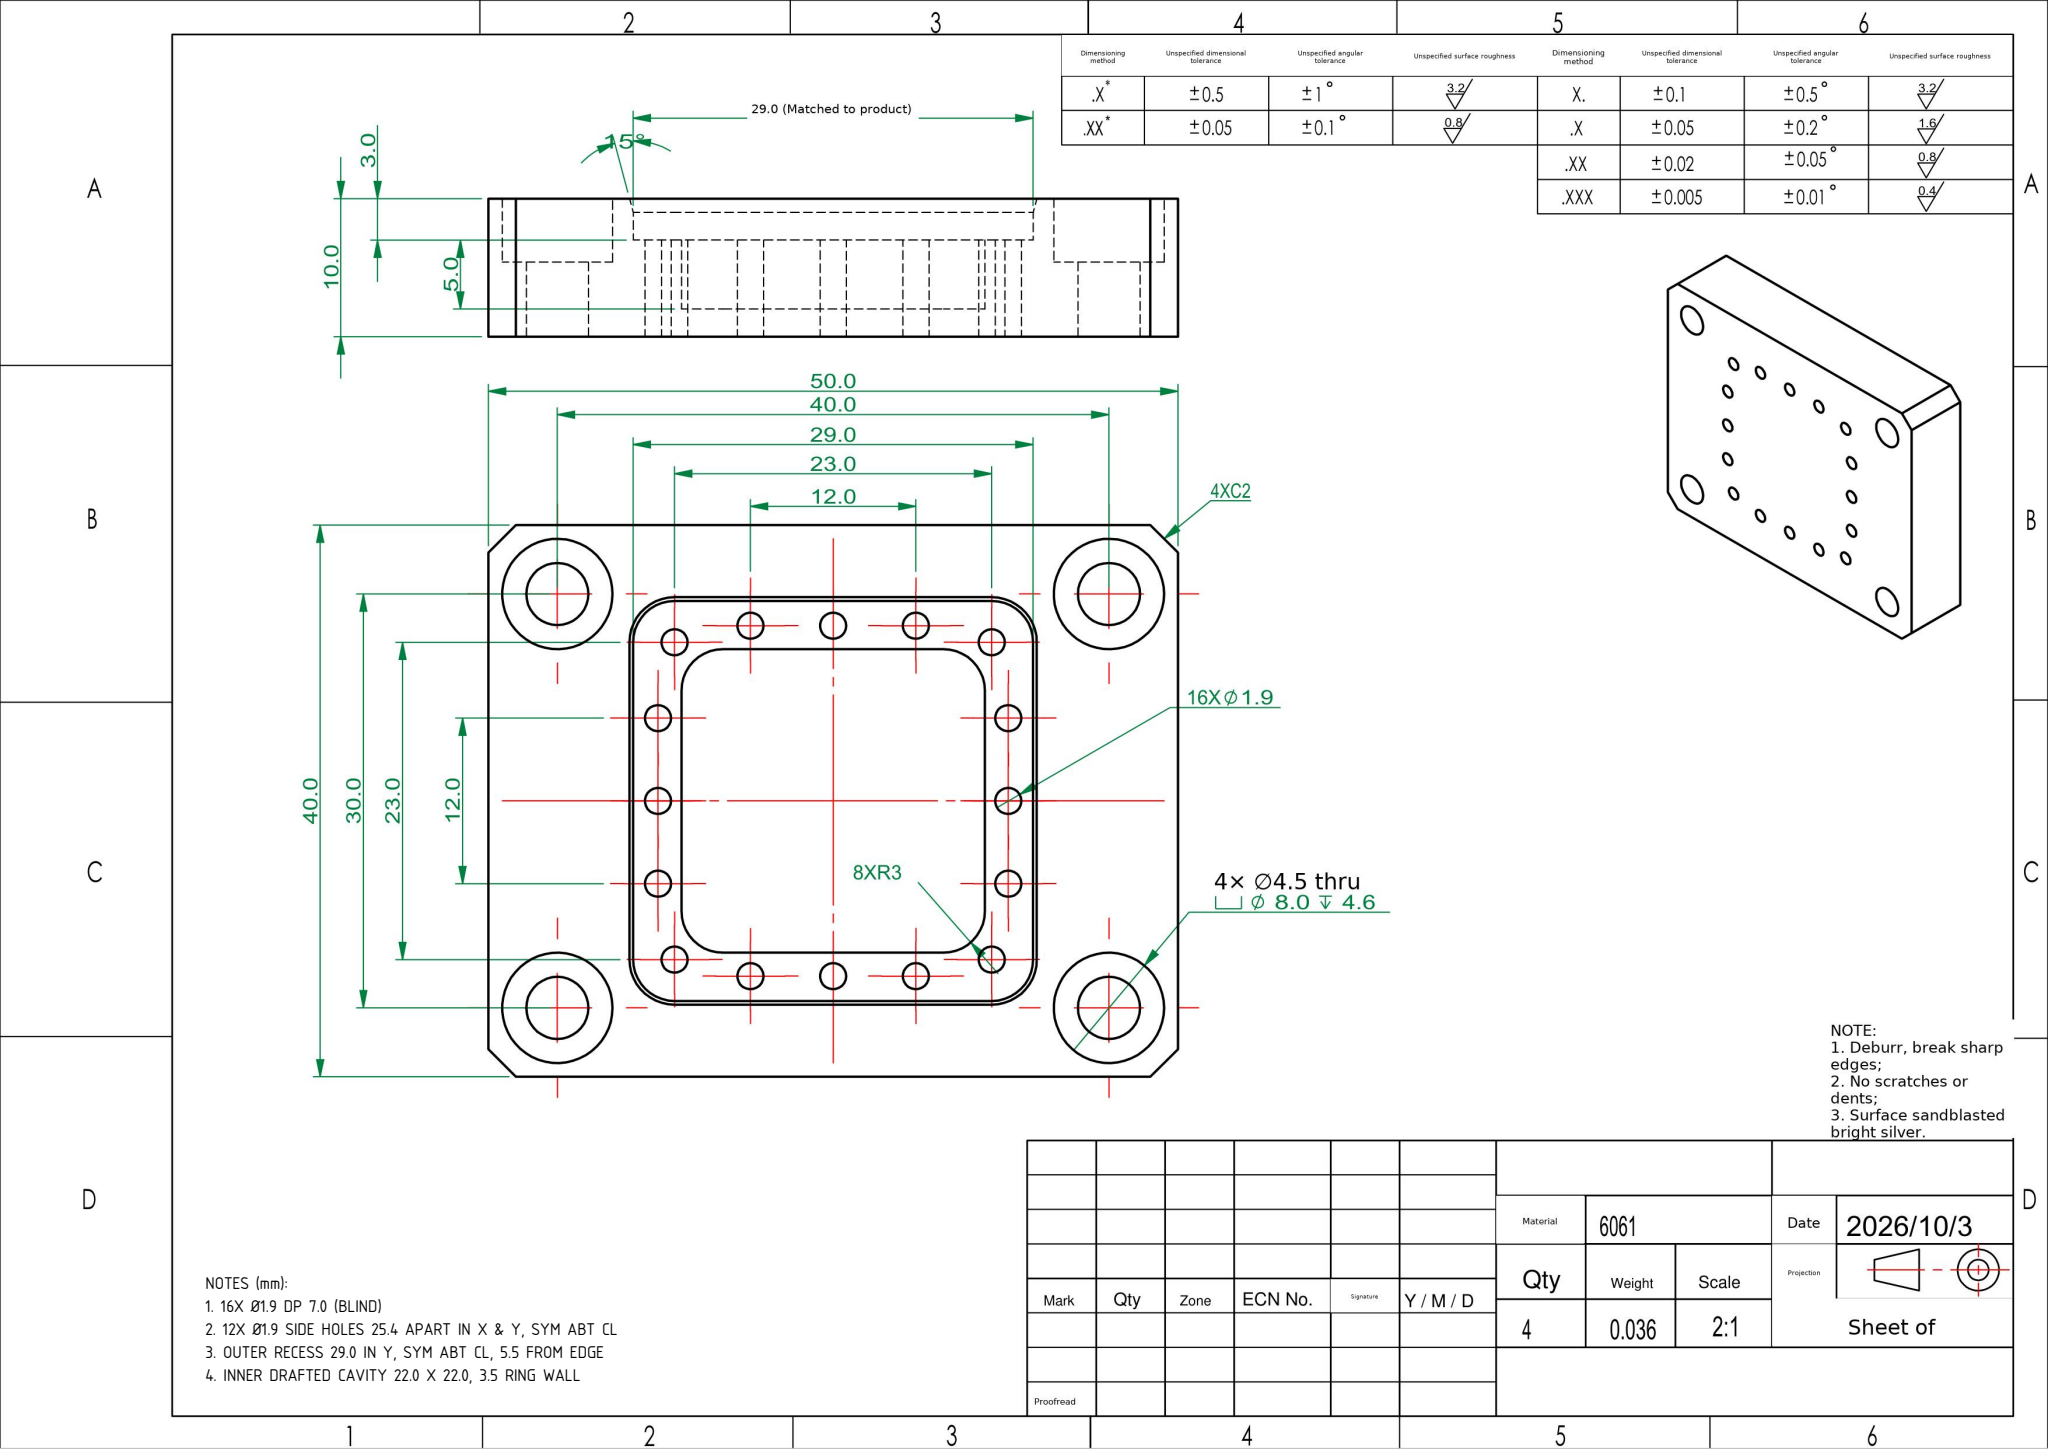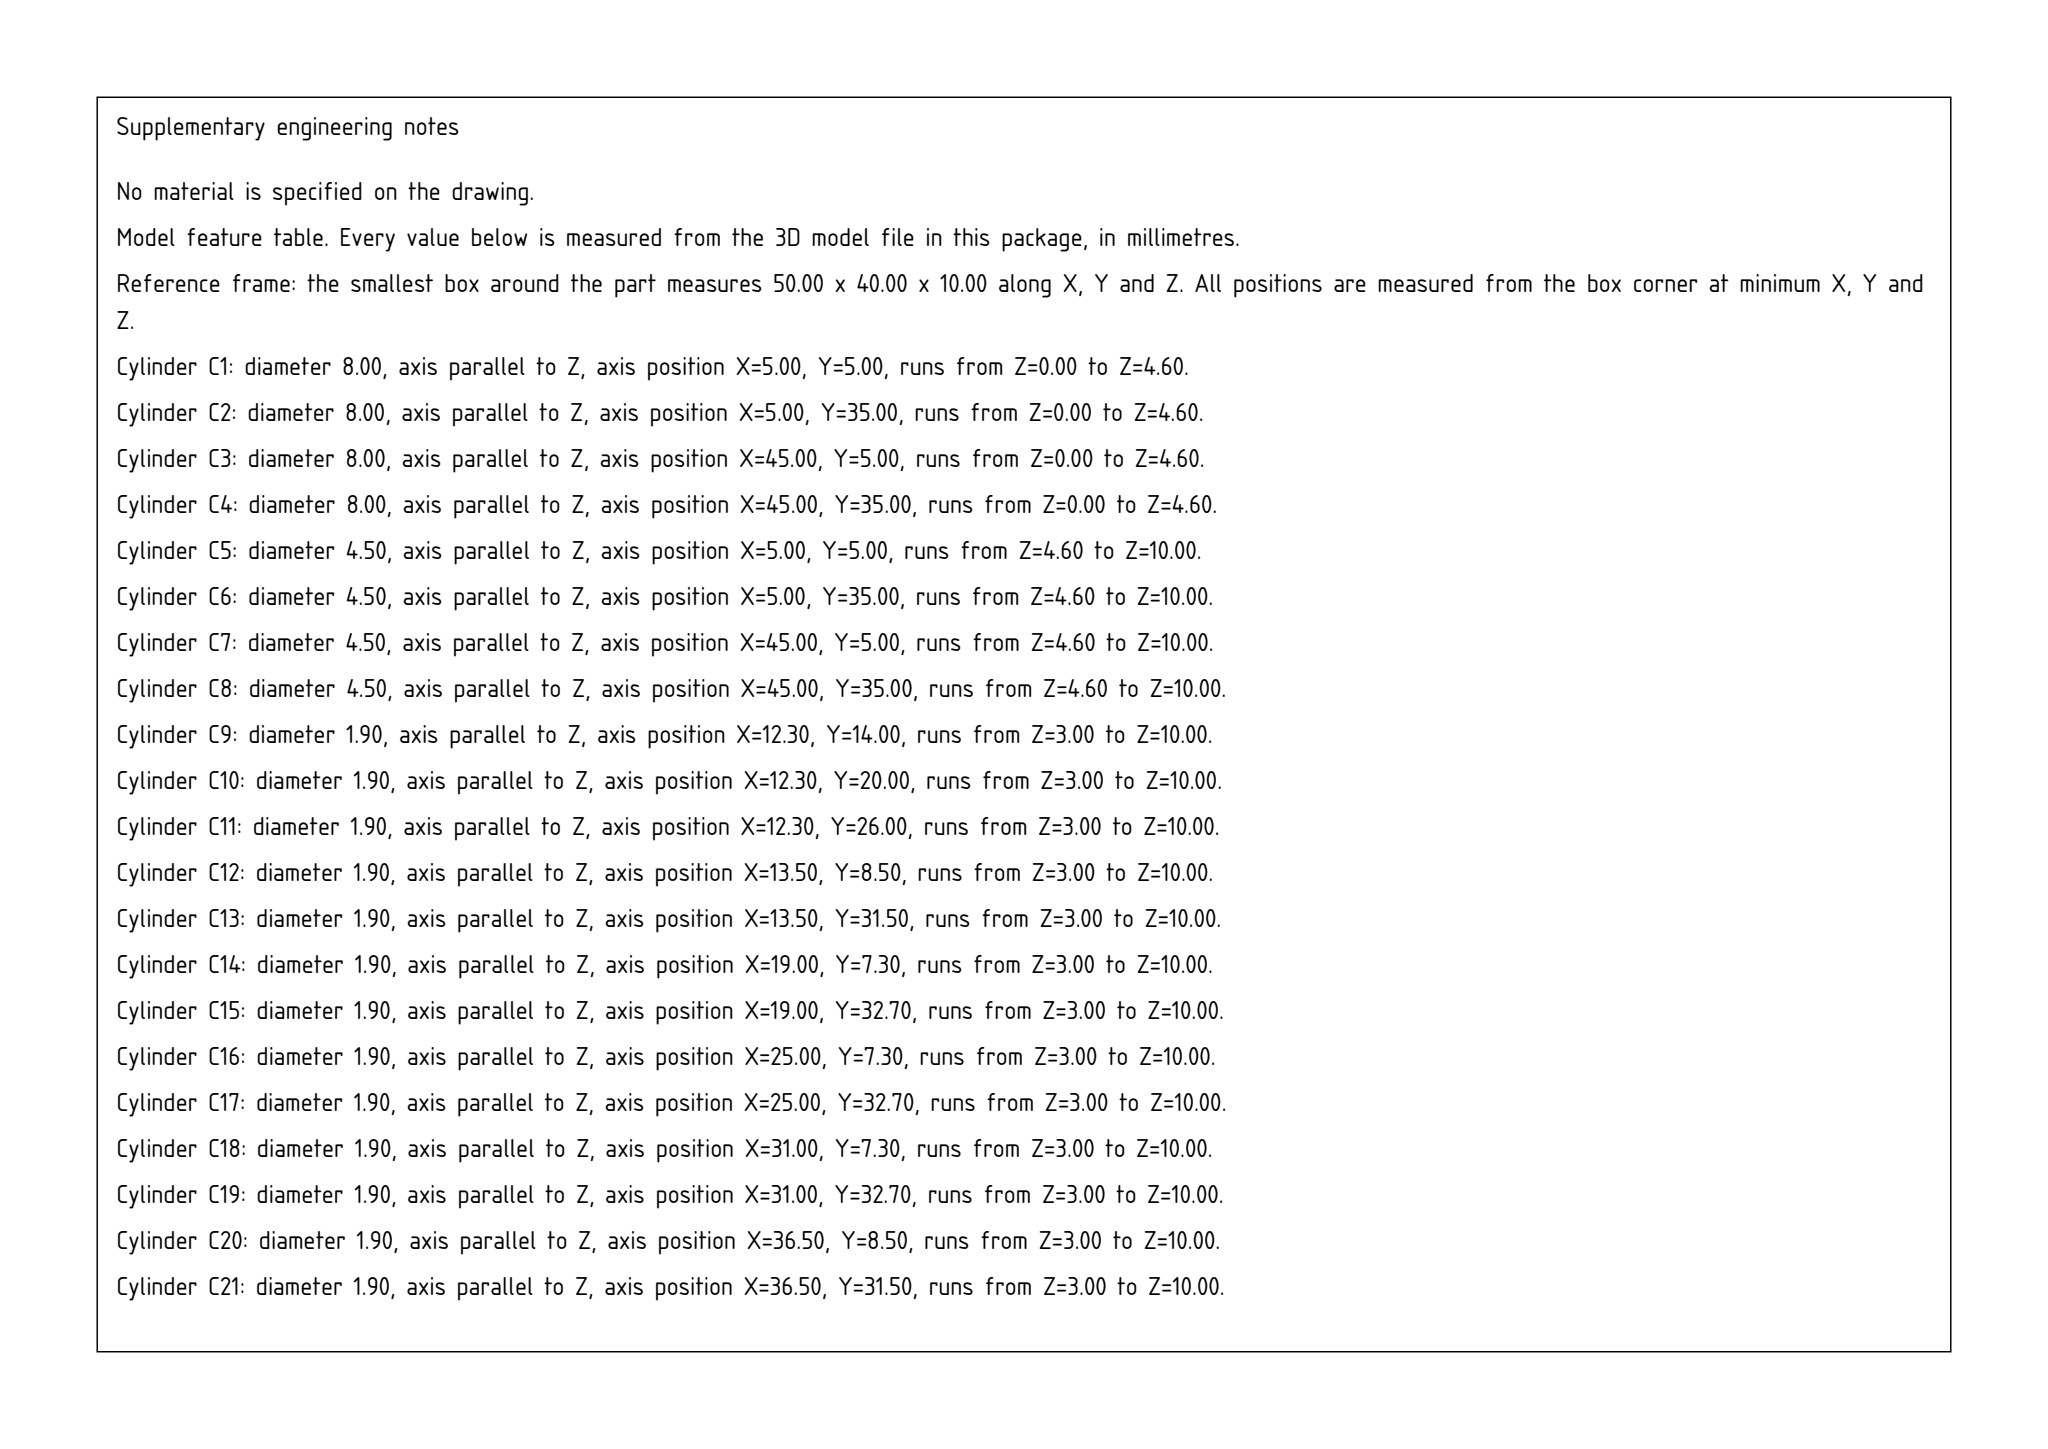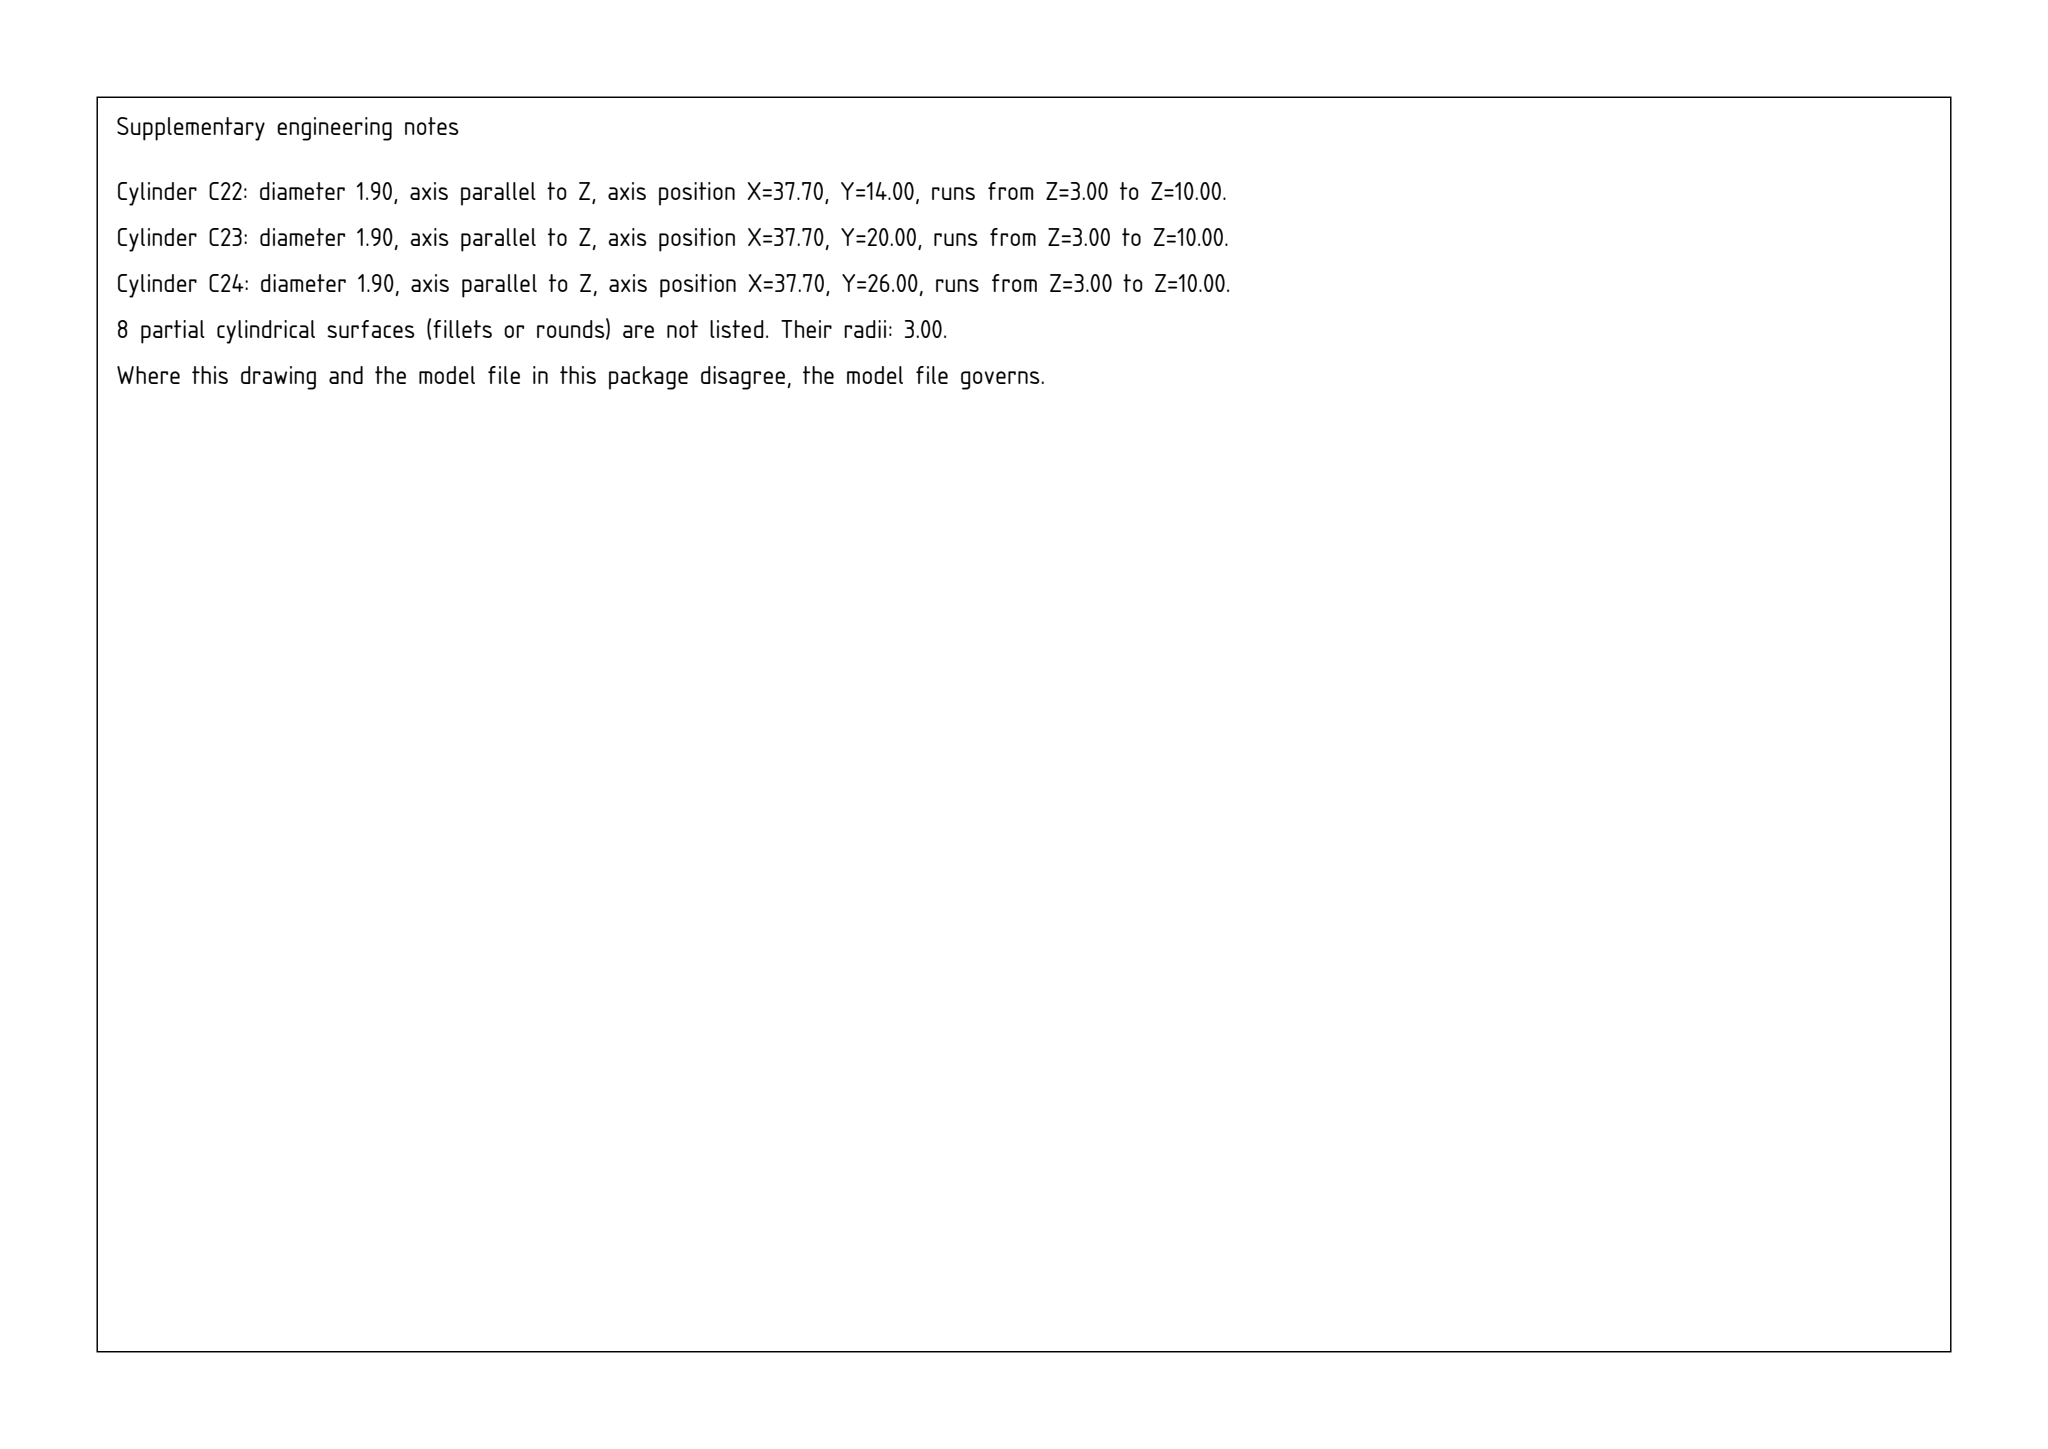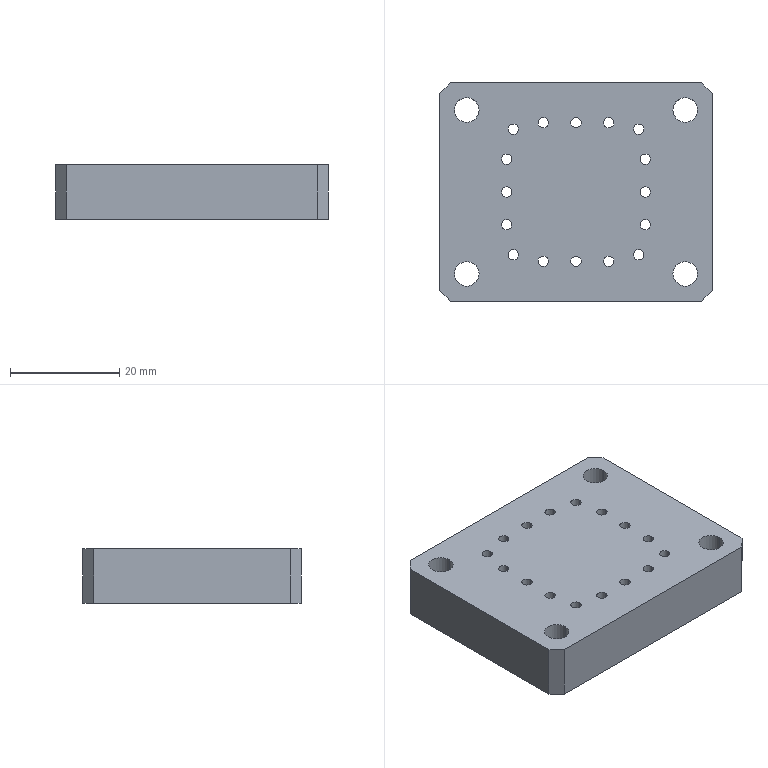Part | SolidWorks | mm | 1 solid | 88 faces | box 50 x 40 x 10 mm | volume 13438 mm3 | cylinder 56 | plane 28 | cone 4 | commonest cylinder face diameters 1.9 x32 8 x8 4.5 x8 6 x8
Drawing notes:
16X Ø1.9 DP 7.0 (BLIND) | from the solid: cylinders dia 1.9, axis z, length 7.0, 16 places
12X Ø1.9 SIDE HOLES 25.4 APART IN X & Y, SYM ABT CL | from the solid: x=12.3/37.7 and y=7.3/32.7 on 50.0 x 40.0 bbox -> 25.4 spans, centered
OUTER RECESS 29.0 IN Y, SYM ABT CL, 5.5 FROM EDGE | from the solid: y planes 5.5 and 34.5 of 40.0 width -> 29.0
INNER DRAFTED CAVITY 22.0 X 22.0, 3.5 RING WALL | from the solid: x planes 14.0/36.0 and y planes 9.0/31.0 -> 22.0; 14.0-10.5=3.5 wall
build123d program:
from build123d import *
from OCP.BRepFilletAPI import BRepFilletAPI_MakeChamfer

# Parameters (mm, degrees)
SKETCH1_W                                         = 50
SKETCH1_H                                         = 40
BOSS_EXTRUDE1_DEPTH                               = 10
SKETCH2_W                                         = 29
SKETCH2_H                                         = 29
CUT_EXTRUDE1_DEPTH                                = 3
SKETCH6_W                                         = 22
SKETCH6_H                                         = 22
CUT_EXTRUDE3_DEPTH                                = 5
HOLE_SIZE_ACCORDING_TO_HEXAGON_SOCKET_D           = 4.5
HOLE_SIZE_ACCORDING_TO_HEXAGON_SOCKET_CBORE_D     = 8
HOLE_SIZE_ACCORDING_TO_HEXAGON_SOCKET_CBORE_DEPTH = 4.6
FILLET1_R                                         = 3
F_1_9_1_9_DIAMETER_HOLE4_D                        = 1.9
F_1_9_1_9_DIAMETER_HOLE4_DEPTH                    = 10
F_1_9_1_9_DIAMETER_HOLE4_TIP                      = 0.5708
F_1_9_1_9_DIAMETER_HOLE5_D                        = 1.9
F_1_9_1_9_DIAMETER_HOLE5_DEPTH                    = 10
F_1_9_1_9_DIAMETER_HOLE5_TIP                      = 0.5708
CHAMFER1_SIZE                                     = 2
CHAMFER2_SIZE                                     = 1
CHAMFER2_SIZE2                                    = 0.2679


with BuildPart() as part:
    # Sketch1 → Boss-Extrude1 (new body)
    with BuildSketch(Plane.XY):
        Rectangle(SKETCH1_W, SKETCH1_H)
    extrude(amount=BOSS_EXTRUDE1_DEPTH)

    # Sketch2 → Cut-Extrude1 (cut)
    with BuildSketch(Plane(origin=(0, 0, 0), x_dir=(-1, 0, 0), z_dir=(0, 0, -1))):
        Rectangle(SKETCH2_W, SKETCH2_H)
    extrude(amount=-CUT_EXTRUDE1_DEPTH, mode=Mode.SUBTRACT)

    # Sketch6 → Cut-Extrude3 (cut)
    with BuildSketch(Plane(origin=(0, 0, 3), x_dir=(-1, 0, 0), z_dir=(0, 0, -1))):
        Rectangle(SKETCH6_W, SKETCH6_H)
    extrude(amount=-CUT_EXTRUDE3_DEPTH, mode=Mode.SUBTRACT)

    # Hole Size _ according to_ Hexagon Socket (through all)
    with Locations(Plane(origin=(-20, 15, 0), x_dir=(-1, 0, 0), z_dir=(0, 0, -1))):
        with Locations((0, 0), (-40, 0), (-40, -30), (0, -30)):
            CounterBoreHole(HOLE_SIZE_ACCORDING_TO_HEXAGON_SOCKET_D / 2, HOLE_SIZE_ACCORDING_TO_HEXAGON_SOCKET_CBORE_D / 2, HOLE_SIZE_ACCORDING_TO_HEXAGON_SOCKET_CBORE_DEPTH)

    # Fillet1
    fillet1_edges = [part.edges().sort_by_distance(p)[0] for p in [
        (-14.5, 14.5, 1.5),
        (-14.5, -14.5, 1.5),
        (14.5, -14.5, 1.5),
        (14.5, 14.5, 1.5),
        (11, -11, 5.5),
        (11, 11, 5.5),
        (-11, 11, 5.5),
        (-11, -11, 5.5),
    ]]
    fillet(fillet1_edges, radius=FILLET1_R)

    # 1.9 _1.9_ Diameter Hole4
    with Locations(Plane(origin=(11.5, 11.5, 3), x_dir=(-1, 0, 0), z_dir=(0, 0, -1))):
        with Locations((0, 0), (23, 0), (23, -23), (0, -23)):
            Hole(F_1_9_1_9_DIAMETER_HOLE4_D / 2, depth=F_1_9_1_9_DIAMETER_HOLE4_DEPTH)
            with Locations((0, 0, -(F_1_9_1_9_DIAMETER_HOLE4_DEPTH + F_1_9_1_9_DIAMETER_HOLE4_TIP / 2))):  # 118° drill point
                Cone(0, F_1_9_1_9_DIAMETER_HOLE4_D / 2, F_1_9_1_9_DIAMETER_HOLE4_TIP, mode=Mode.SUBTRACT)

    # 1.9 _1.9_ Diameter Hole5
    with Locations(Plane(origin=(-6, 12.7, 3), x_dir=(-1, 0, 0), z_dir=(0, 0, -1))):
        with Locations((0, 0), (0, -25.4), (-18.7, -12.7), (6.7, -12.7), (-12, 0), (-6, 0), (6.7, -6.7), (6.7, -18.7), (-6, -25.4), (-12, -25.4), (-18.7, -18.7), (-18.7, -6.7)):
            Hole(F_1_9_1_9_DIAMETER_HOLE5_D / 2, depth=F_1_9_1_9_DIAMETER_HOLE5_DEPTH)
            with Locations((0, 0, -(F_1_9_1_9_DIAMETER_HOLE5_DEPTH + F_1_9_1_9_DIAMETER_HOLE5_TIP / 2))):  # 118° drill point
                Cone(0, F_1_9_1_9_DIAMETER_HOLE5_D / 2, F_1_9_1_9_DIAMETER_HOLE5_TIP, mode=Mode.SUBTRACT)

    # Chamfer1
    chamfer1_edges = [part.edges().sort_by_distance(p)[0] for p in [
        (25, -20, 5),
        (-25, -20, 5),
        (-25, 20, 5),
        (25, 20, 5),
    ]]
    chamfer(chamfer1_edges, length=CHAMFER1_SIZE)

    # Chamfer2: one chamfer whose edges measure the first distance from different faces: ONE call of the kernel's chamfer builder (chamfer() names one face for all edges)
    chamfer2_edges_1 = [part.edges().sort_by_distance(p)[0] for p in [
        (0, -14.5, 0),
    ]]
    chamfer2_side_1 = [part.faces().sort_by_distance(p)[0] for p in [
        (0, -14.5, 1.5),
    ]]
    chamfer2_edges_2 = [part.edges().sort_by_distance(p)[0] for p in [
        (14.5, 0, 0),
    ]]
    chamfer2_side_2 = [part.faces().sort_by_distance(p)[0] for p in [
        (14.5, 0, 1.5),
    ]]
    chamfer2_edges_3 = [part.edges().sort_by_distance(p)[0] for p in [
        (-14.5, 0, 0),
    ]]
    chamfer2_side_3 = [part.faces().sort_by_distance(p)[0] for p in [
        (-14.5, 0, 1.5),
    ]]
    chamfer2_edges_4 = [part.edges().sort_by_distance(p)[0] for p in [
        (0, 14.5, 0),
    ]]
    chamfer2_side_4 = [part.faces().sort_by_distance(p)[0] for p in [
        (0, 14.5, 1.5),
    ]]
    chamfer2_edges_5 = [part.edges().sort_by_distance(p)[0] for p in [
        (13.621, -13.621, 0),
    ]]
    chamfer2_side_5 = [part.faces().sort_by_distance(p)[0] for p in [
        (13.621, -13.621, 1.5),
    ]]
    chamfer2_edges_6 = [part.edges().sort_by_distance(p)[0] for p in [
        (-13.621, -13.621, 0),
    ]]
    chamfer2_side_6 = [part.faces().sort_by_distance(p)[0] for p in [
        (-13.621, -13.621, 1.5),
    ]]
    chamfer2_edges_7 = [part.edges().sort_by_distance(p)[0] for p in [
        (-13.621, 13.621, 0),
    ]]
    chamfer2_side_7 = [part.faces().sort_by_distance(p)[0] for p in [
        (-13.621, 13.621, 1.5),
    ]]
    chamfer2_edges_8 = [part.edges().sort_by_distance(p)[0] for p in [
        (13.621, 13.621, 0),
    ]]
    chamfer2_side_8 = [part.faces().sort_by_distance(p)[0] for p in [
        (13.621, 13.621, 1.5),
    ]]
    chamfer2 = BRepFilletAPI_MakeChamfer(part.part.solid().wrapped)
    for e in chamfer2_edges_1:
        chamfer2.Add(CHAMFER2_SIZE, CHAMFER2_SIZE2, e.wrapped, chamfer2_side_1[0].wrapped)  # the first distance lies on this face
    for e in chamfer2_edges_2:
        chamfer2.Add(CHAMFER2_SIZE, CHAMFER2_SIZE2, e.wrapped, chamfer2_side_2[0].wrapped)  # the first distance lies on this face
    for e in chamfer2_edges_3:
        chamfer2.Add(CHAMFER2_SIZE, CHAMFER2_SIZE2, e.wrapped, chamfer2_side_3[0].wrapped)  # the first distance lies on this face
    for e in chamfer2_edges_4:
        chamfer2.Add(CHAMFER2_SIZE, CHAMFER2_SIZE2, e.wrapped, chamfer2_side_4[0].wrapped)  # the first distance lies on this face
    for e in chamfer2_edges_5:
        chamfer2.Add(CHAMFER2_SIZE, CHAMFER2_SIZE2, e.wrapped, chamfer2_side_5[0].wrapped)  # the first distance lies on this face
    for e in chamfer2_edges_6:
        chamfer2.Add(CHAMFER2_SIZE, CHAMFER2_SIZE2, e.wrapped, chamfer2_side_6[0].wrapped)  # the first distance lies on this face
    for e in chamfer2_edges_7:
        chamfer2.Add(CHAMFER2_SIZE, CHAMFER2_SIZE2, e.wrapped, chamfer2_side_7[0].wrapped)  # the first distance lies on this face
    for e in chamfer2_edges_8:
        chamfer2.Add(CHAMFER2_SIZE, CHAMFER2_SIZE2, e.wrapped, chamfer2_side_8[0].wrapped)  # the first distance lies on this face
    add(Compound.cast(chamfer2.Shape()), mode=Mode.REPLACE)


solid = part.part